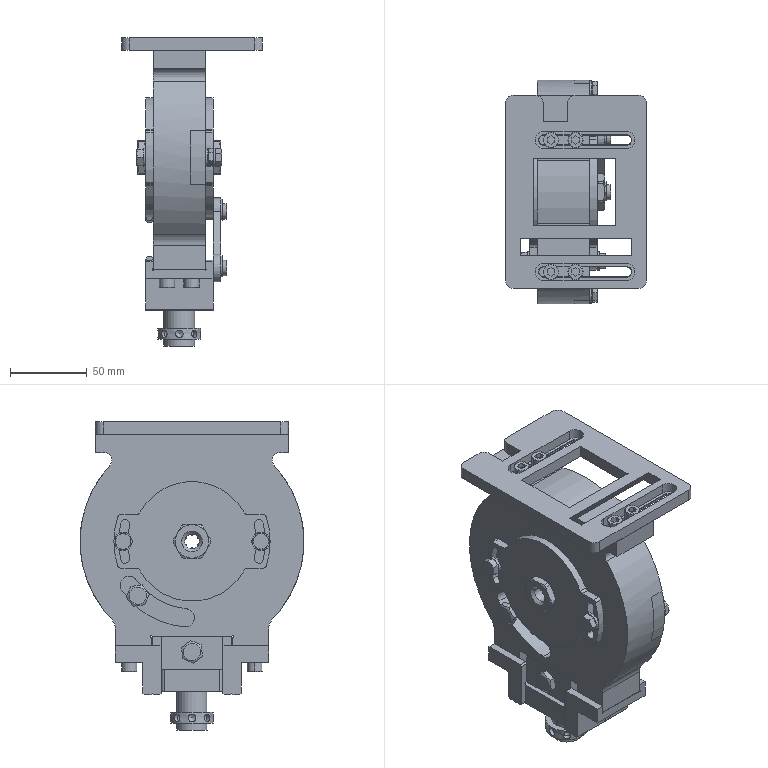Assembly | NX | mm | 53 component files | 53 solids | 1192 faces | box 92 x 146 x 201.11 mm | volume 761396 mm3 | plane 660 | cylinder 321 | cone 157 | torus 48 | sphere 6 | commonest cylinder face diameters 6 x64 10 x39 20 x28 4 x26 1 x22 12 x14 8 x12 24.5 x12
Bill of materials:
unnamed part 1 | 1 |  | Hollow flanged bushing-like part: a hexagonal flange with a reduced-diameter neck/undercut, then a larger cylindrical sleeve with a chamfered free end; a round through-bore runs along the axis.
unnamed part 2 | 1 |  | Thin flat rectangular plate with rounded outer corners, a rectangular notch at one end edge, two parallel rounded-end slots, one large square cutout and one long rectangular cutout.
unnamed part 3 | 1 |  | Prismatic block with rectangular tabs sticking out of two opposite faces, a single round through-hole in one side face, and a lower base section with a channel and hooked or L-shaped retaining lips along the bottom.
unnamed part 4 | 1 |  | Cylindrical tube with an outer radial collar/flange; the collar rim has several evenly spaced radial holes that appear to be blind holes with conical bottoms.
unnamed part 5 | 6 |  | Solid prismatic block with a polygonal (partly hexagonal/angled) profile containing a large open C-shaped recess with inward-stepped lips; one end face carries two small raised rail or catch features and a small rounded protrusion appears on the profile edge.
unnamed part 6 | 2 |  | Flat open split ring of uniform thickness with two extended lugs at the gap, each lug having a small round hole; looks like an external retaining-ring-style shape.
unnamed part 7 | 1 |  | Flanged washer or bushing: a wide thin circular disc with a chamfered top edge and a shorter, smaller-diameter cylindrical hub underneath; a small central through-hole with a slight edge chamfer.
unnamed part 8 | 2 |  | Thin circular plate with a short cylindrical boss on one face, a central round through-hole, and two opposite flat tabs each with an arc-shaped elongated slot.
unnamed part 9 | 2 |  | Block with an L-shaped side profile and a U/H-shaped top layout: a flat top web with an obround slot and a rectangular notch, two raised side rails with small corner relief holes, and downward legs with chamfered corners and a small V-notch at the bottom.
unnamed part 10 | 2 |  | Pin with a hexagonal head and a long plain cylindrical shank; a narrow circumferential groove sits near the chamfered free end.
unnamed part 11 | 6 |  | Stepped pin with a domed, rounded head, a main cylindrical shank, a reduced-diameter neck groove, and a short chamfered end section.
unnamed part 12 | 4 |  | Cap-screw-like solid: a cylindrical head of larger diameter and a smaller plain cylindrical shank with a chamfered tip; head end shows a concentric recess or step.
unnamed part 13 | 1 |  | Flat circular ring plate with a large central hexagonal opening with rounded corners and six small round through-holes evenly spaced around the outer band.
unnamed part 14 | 1 |  | Thin flat circular plate with a central rounded hexagonal opening, two opposite rectangular side tabs, two curved arc slots, and four small round holes in a line across the middle (two in the tabs, two next to the hex opening).
unnamed part 15 | 1 |  | Flat link bar: a straight strap with a rounded boss at each end, each boss pierced by one round through-hole.
unnamed part 16 | 1 |  | Hexagonal block with rounded corners and a central through-bore. The bore has a large shallow counterbore or recess on one hex face, and smaller cross-holes run radially through several flat side faces into the bore.
unnamed part 17 | 1 |  | Flanged bushing or sleeve: a cylindrical body with a chamfered free end, a smaller-diameter neck or undercut, and a hexagonal flange with chamfered corners, with a central through-bore that is chamfered or countersunk at the flange end.
unnamed part 18 | 5 |  | Socket-head cap-screw-like part: a cylindrical head with a hexagonal socket recess and a plain cylindrical shank with a chamfered tip.
unnamed part 19 | 1 |  | Bracket plate: a roughly circular body with a flat rectangular bar along the top carrying four small holes, two rectangular feet at the bottom, a central rounded hexagonal opening, one curved arc slot, small holes on the horizontal centerline, and stepped or layered thickness with a groove visible in the side view.
unnamed part 20 | 6 |  | Plain flat annular ring or washer with a central round hole; the bore edge appears slightly chamfered on at least one side.
unnamed part 21 | 2 |  | Hex-head bolt-like part with a long plain cylindrical shank, a chamfered tip, and a small round collar or washer face under the hex head.
unnamed part 22 | 4 |  | Hex-head bolt-like part with a shorter plain cylindrical shank, a fillet at the head-shank junction, and a chamfered tip.
unnamed part 23 | 1 |  | Thick flat washer or spacer ring with chamfered outer edges on both faces and chamfered bore edges.
Mates:
1. fix | Mounting_Bracket 1 component
2. touch align | Housing 1 face | Mounting_Bracket 1 face
3. center | Mounting_Bracket 1 face | Mounting_Bracket 1 face | Housing 1 face
4. touch align | SHCS_M6x12 5 face | Housing 1 face
5. touch align | Mounting_Bracket 1 face | SHCS_M6x12 5 face
6. touch align | SHCS_M6x12 4 face | Housing 1 face
7. touch align | Mounting_Bracket 1 face | SHCS_M6x12 4 face
8. bond | Mounting_Bracket 1 component | assembly component
9. bond | SHCS_M6x12 5 component | assembly component
10. bond | SHCS_M6x12 4 component | assembly component
11. bond | SHCS_M6x12 3 component | assembly component
12. bond | SHCS_M6x12 2 component | assembly component
13. linear | assembly datumaxis | assembly cartesiancoordinatesystem | assembly cartesiancoordinatesystem
14. linear | assembly datumaxis | assembly cartesiancoordinatesystem | assembly cartesiancoordinatesystem
15. touch align | Six_Side_Body 1 face | Housing 1 face
16. parallel | Six_Side_Body 1 face | Housing 1 face
17. center | Clamping_Block 6 face | Clamping_Block 6 face | Connecting_Shaft 6 face
18. center | Clamping_Block 6 face | Clamping_Block 6 face | Connecting_Shaft 6 face
19. touch align | Connecting_Shaft 6 face | Clamping_Block 6 face
20. bond | Six_Side_Body 1 component | assembly component
21. bond | Connecting_Shaft 6 component | assembly component
22. bond | Clamping_Block 6 component | assembly component
23. bond | Connecting_Shaft 5 component | assembly component
24. bond | Clamping_Block 5 component | assembly component
25. bond | Connecting_Shaft 4 component | assembly component
26. bond | Clamping_Block 4 component | assembly component
27. circular | assembly datumaxis | assembly cartesiancoordinatesystem | assembly cartesiancoordinatesystem | assembly cartesiancoordinatesystem | assembly cartesiancoordinatesystem | assembly cartesiancoordinatesystem | assembly cartesiancoordinatesystem
28. circular | assembly datumaxis | assembly cartesiancoordinatesystem | assembly cartesiancoordinatesystem | assembly cartesiancoordinatesystem | assembly cartesiancoordinatesystem | assembly cartesiancoordinatesystem | assembly cartesiancoordinatesystem
29. bond | Connecting_Shaft 3 component | assembly component
30. bond | Clamping_Block 3 component | assembly component
31. bond | Connecting_Shaft 2 component | assembly component
32. bond | Clamping_Block 2 component | assembly component
33. bond | Connecting_Shaft 1 component | assembly component
34. bond | Clamping_Block 1 component | assembly component
35. parallel | Housing 1 face | Mounting_Bracket 1 face
36. touch align | Connecting_Shaft 6 face | Six_Side_Body 1 face
37. parallel | Clamping_Block 6 face | Mounting_Bracket 1 face
38. touch align | Guide_Block 2 face | Housing 1 face
39. touch align | Guide_Block 2 face | Housing 1 face
40. touch align | Guide_Block 2 face | Housing 1 face
41. touch align | Housing 1 face | Guide_Block 1 face
42. touch align | Guide_Block 1 face | Housing 1 face
43. touch align | Guide_Block 1 face | Housing 1 face
44. touch align | SHCS_M6x20 4 | Housing 1 face
45. touch align | Guide_Block 2 face | SHCS_M6x20 4
46. touch align | SHCS_M6x20 3 face | Housing 1 face
47. touch align | SHCS_M6x20 3 face | Guide_Block 2 face
48. touch align | SHCS_M6x20 2 | Housing 1 face
49. touch align | SHCS_M6x20 2 | Guide_Block 1 face
50. touch align | SHCS_M6x20 1 | Housing 1 face
51. touch align | SHCS_M6x20 1 | Guide_Block 1 face
52. concentric | Housing_Cover 1 arc | Housing 1 edge
53. parallel | Housing_Cover 1 face | Housing 1 face
54. center | Housing_Cover 1 face | Housing 1 face | Connecting_Shaft 6 face
55. concentric | End_Cap 2 edge | Housing 1 edge
56. parallel | End_Cap 2 face | Mounting_Bracket 1 face
57. concentric | Six_Side_Body 1 edge | End_Cap 1 edge
58. parallel | End_Cap 1 face | Mounting_Bracket 1 face
59. concentric | Inlet_Screw 1 edge | End_Cap 1 edge
60. parallel | Inlet_Screw 1 face | Mounting_Bracket 1 face
61. concentric | End_Cap 2 edge | Outlet_Screw 1 edge
62. parallel | Outlet_Screw 1 face | Mounting_Bracket 1 face
63. touch align | Turntable 1 face | Housing 1 face
64. center | Turntable 1 face | Turntable 1 face | Six_Side_Body 1 face | Six_Side_Body 1 face
65. concentric | Washer_M6 6 arc | Housing_Cover 1 edge
66. concentric | Washer_M6 5 arc | Housing_Cover 1 edge
67. concentric | Hex_Bolt_M6x25_FT 1 | Washer_M6 6
68. concentric | Washer_M6 5 edge | Hex_Bolt_M6x25_FT 2 edge
69. parallel | Slider 1 face | Housing 1 face
70. center | Slider 1 face | Slider 1 face | Guide_Block 2 face | Guide_Block 1 face
71. center | Slider 1 face | Slider 1 face | Guide_Block 2 face | Guide_Block 2 face
72. touch align | Slider 1 face | Clamp_Block 1 face
73. center | Slider 1 face | Slider 1 face | Clamp_Block 1 face
74. center | Slider 1 face | Slider 1 face | Clamp_Block 1 face
75. touch align | Eight_Hole_Clamp_Block 1 face | Clamp_Block 1 face
76. touch align | Clamp_Block 1 face | Eight_Hole_Clamp_Block 1 face
77. concentric | Stopper 1 edge | Clamp_Block 1 edge
78. concentric | SHCS_M6x12 1 edge | Stopper 1 edge
79. touch align | Washer_M6 4 | Housing_Cover 1 face
80. touch align | Washer_M6 4 | End_Cap 2 face
81. touch align | Washer_M6 3 | Housing_Cover 1 face
82. touch align | Washer_M6 3 | End_Cap 2 face
83. concentric | Hex_Bolt_M6x16_FT_C 4 | Washer_M6 4
84. concentric | Hex_Bolt_M6x16_FT_C 3 | Washer_M6 3
85. touch align | End_Cap 1 face | Washer_M6 2 face
86. touch align | Washer_M6 2 face | Housing 1 face
87. touch align | End_Cap 1 face | Washer_M6 1
88. touch align | Washer_M6 1 | Housing 1 face
89. concentric | Hex_Bolt_M6x16_FT_C 2 edge | Washer_M6 2 edge
90. concentric | Hex_Bolt_M6x16_FT_C 1 | Washer_M6 1
91. concentric | Rotating_Shaft 2 | Slider 1 edge
92. touch align | Rotating_Shaft 1 face | Turntable 1 face
93. touch align | Rotating_Shaft 1 face | Housing 1 face
94. touch align | Connecting_Rod 1 face | Rotating_Shaft 2
95. touch align | Connecting_Rod 1 face | Rotating_Shaft 1 face
96. touch align | Connecting_Rod 1 face | Guide_Block 2 face
97. concentric | Retaining_Ring 2 arc | Connecting_Rod 1 edge
98. concentric | Retaining_Ring 1 arc | Connecting_Rod 1 edge